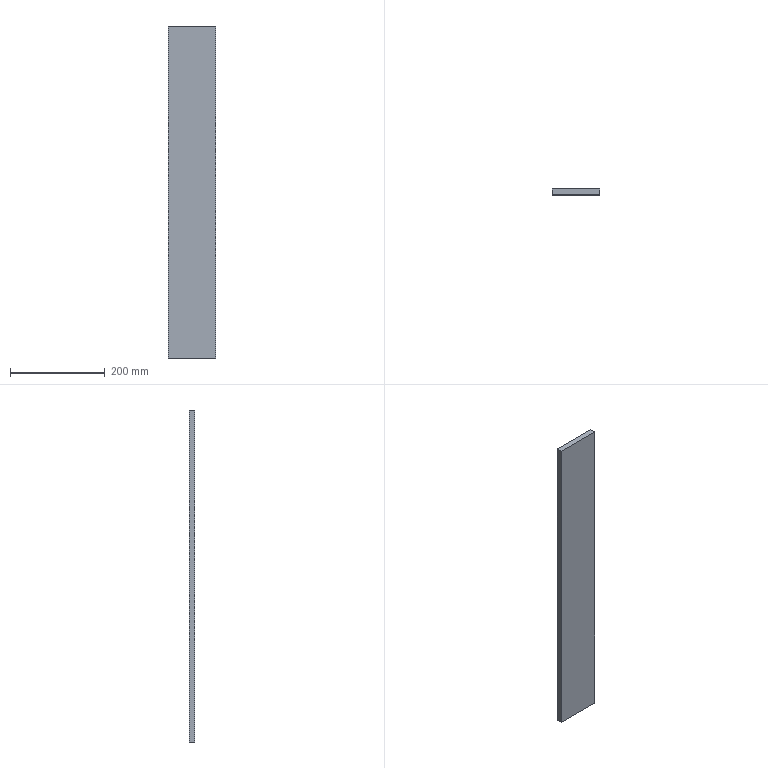Component | NX | CHAPA_INTERNA | 1 solid | 6 faces | box 100 x 12 x 700 mm | volume 840000 mm3 | plane 6
STEP:
#1=CARTESIAN_POINT('',(0.,0.,0.));
#2=DIRECTION('',(0.,0.,1.));
#3=DIRECTION('',(1.,0.,0.));
#4=AXIS2_PLACEMENT_3D('',#1,#2,#3);
#5=CARTESIAN_POINT('',(0.,-22.8,700.));
#6=VERTEX_POINT('',#5);
#7=CARTESIAN_POINT('',(0.,-22.8,0.));
#8=VERTEX_POINT('',#7);
#9=CARTESIAN_POINT('',(0.,-22.8,700.));
#10=DIRECTION('',(0.,0.,-1.));
#11=VECTOR('',#10,1.);
#12=LINE('',#9,#11);
#13=CARTESIAN_POINT('',(0.,-34.8,700.));
#14=DIRECTION('',(1.,0.,0.));
#15=DIRECTION('',(0.,0.,-1.));
#16=AXIS2_PLACEMENT_3D('',#13,#14,#15);
#17=PLANE('',#16);
#18=CARTESIAN_POINT('',(0.,12.));
#19=DIRECTION('',(1.,0.));
#20=VECTOR('',#19,1.);
#21=LINE('',#18,#20);
#22=(GEOMETRIC_REPRESENTATION_CONTEXT(2)PARAMETRIC_REPRESENTATION_CONTEXT()REPRESENTATION_CONTEXT('',''));
#23=DEFINITIONAL_REPRESENTATION('',(#21),#22);
#24=PCURVE('',#17,#23);
#25=CARTESIAN_POINT('',(0.,-22.8,0.));
#26=DIRECTION('',(0.,-1.,0.));
#27=DIRECTION('',(0.,0.,-1.));
#28=AXIS2_PLACEMENT_3D('',#25,#26,#27);
#29=PLANE('',#28);
#30=CARTESIAN_POINT('',(-700.,-0.));
#31=DIRECTION('',(1.,0.));
#32=VECTOR('',#31,1.);
#33=LINE('',#30,#32);
#34=(GEOMETRIC_REPRESENTATION_CONTEXT(2)PARAMETRIC_REPRESENTATION_CONTEXT()REPRESENTATION_CONTEXT('',''));
#35=DEFINITIONAL_REPRESENTATION('',(#33),#34);
#36=PCURVE('',#29,#35);
#37=SURFACE_CURVE('',#12,(#24,#36),.PCURVE_S1.);
#38=EDGE_CURVE('',#6,#8,#37,.T.);
#39=ORIENTED_EDGE('',*,*,#38,.T.);
#40=CARTESIAN_POINT('',(0.,-34.8,0.));
#41=VERTEX_POINT('',#40);
#42=CARTESIAN_POINT('',(0.,-34.8,0.));
#43=DIRECTION('',(0.,1.,0.));
#44=VECTOR('',#43,1.);
#45=LINE('',#42,#44);
#46=CARTESIAN_POINT('',(700.,0.));
#47=DIRECTION('',(0.,1.));
#48=VECTOR('',#47,1.);
#49=LINE('',#46,#48);
#50=(GEOMETRIC_REPRESENTATION_CONTEXT(2)PARAMETRIC_REPRESENTATION_CONTEXT()REPRESENTATION_CONTEXT('',''));
#51=DEFINITIONAL_REPRESENTATION('',(#49),#50);
#52=PCURVE('',#17,#51);
#53=CARTESIAN_POINT('',(0.,-34.8,0.));
#54=DIRECTION('',(-0.,0.,1.));
#55=DIRECTION('',(1.,0.,0.));
#56=AXIS2_PLACEMENT_3D('',#53,#54,#55);
#57=PLANE('',#56);
#58=CARTESIAN_POINT('',(0.,0.));
#59=DIRECTION('',(0.,1.));
#60=VECTOR('',#59,1.);
#61=LINE('',#58,#60);
#62=(GEOMETRIC_REPRESENTATION_CONTEXT(2)PARAMETRIC_REPRESENTATION_CONTEXT()REPRESENTATION_CONTEXT('',''));
#63=DEFINITIONAL_REPRESENTATION('',(#61),#62);
#64=PCURVE('',#57,#63);
#65=SURFACE_CURVE('',#45,(#52,#64),.PCURVE_S1.);
#66=EDGE_CURVE('',#41,#8,#65,.T.);
#67=ORIENTED_EDGE('',*,*,#66,.F.);
#68=CARTESIAN_POINT('',(0.,-34.8,700.));
#69=VERTEX_POINT('',#68);
#70=CARTESIAN_POINT('',(0.,-34.8,700.));
#71=DIRECTION('',(0.,0.,-1.));
#72=VECTOR('',#71,1.);
#73=LINE('',#70,#72);
#74=CARTESIAN_POINT('',(0.,0.));
#75=DIRECTION('',(1.,0.));
#76=VECTOR('',#75,1.);
#77=LINE('',#74,#76);
#78=(GEOMETRIC_REPRESENTATION_CONTEXT(2)PARAMETRIC_REPRESENTATION_CONTEXT()REPRESENTATION_CONTEXT('',''));
#79=DEFINITIONAL_REPRESENTATION('',(#77),#78);
#80=PCURVE('',#17,#79);
#81=CARTESIAN_POINT('',(0.,-34.8,0.));
#82=DIRECTION('',(0.,-1.,0.));
#83=DIRECTION('',(0.,0.,-1.));
#84=AXIS2_PLACEMENT_3D('',#81,#82,#83);
#85=PLANE('',#84);
#86=CARTESIAN_POINT('',(-700.,-0.));
#87=DIRECTION('',(1.,0.));
#88=VECTOR('',#87,1.);
#89=LINE('',#86,#88);
#90=(GEOMETRIC_REPRESENTATION_CONTEXT(2)PARAMETRIC_REPRESENTATION_CONTEXT()REPRESENTATION_CONTEXT('',''));
#91=DEFINITIONAL_REPRESENTATION('',(#89),#90);
#92=PCURVE('',#85,#91);
#93=SURFACE_CURVE('',#73,(#80,#92),.PCURVE_S1.);
#94=EDGE_CURVE('',#69,#41,#93,.T.);
#95=ORIENTED_EDGE('',*,*,#94,.F.);
#96=CARTESIAN_POINT('',(0.,-34.8,700.));
#97=DIRECTION('',(0.,1.,0.));
#98=VECTOR('',#97,1.);
#99=LINE('',#96,#98);
#100=CARTESIAN_POINT('',(0.,0.));
#101=DIRECTION('',(0.,1.));
#102=VECTOR('',#101,1.);
#103=LINE('',#100,#102);
#104=(GEOMETRIC_REPRESENTATION_CONTEXT(2)PARAMETRIC_REPRESENTATION_CONTEXT()REPRESENTATION_CONTEXT('',''));
#105=DEFINITIONAL_REPRESENTATION('',(#103),#104);
#106=PCURVE('',#17,#105);
#107=CARTESIAN_POINT('',(100.,-34.8,700.));
#108=DIRECTION('',(0.,0.,-1.));
#109=DIRECTION('',(-1.,0.,0.));
#110=AXIS2_PLACEMENT_3D('',#107,#108,#109);
#111=PLANE('',#110);
#112=CARTESIAN_POINT('',(100.,0.));
#113=DIRECTION('',(0.,1.));
#114=VECTOR('',#113,1.);
#115=LINE('',#112,#114);
#116=(GEOMETRIC_REPRESENTATION_CONTEXT(2)PARAMETRIC_REPRESENTATION_CONTEXT()REPRESENTATION_CONTEXT('',''));
#117=DEFINITIONAL_REPRESENTATION('',(#115),#116);
#118=PCURVE('',#111,#117);
#119=SURFACE_CURVE('',#99,(#106,#118),.PCURVE_S1.);
#120=EDGE_CURVE('',#69,#6,#119,.T.);
#121=ORIENTED_EDGE('',*,*,#120,.T.);
#122=EDGE_LOOP('',(#39,#67,#95,#121));
#123=FACE_BOUND('',#122,.T.);
#124=ADVANCED_FACE('',(#123),#17,.F.);
#125=CARTESIAN_POINT('',(100.,-22.8,0.));
#126=VERTEX_POINT('',#125);
#127=CARTESIAN_POINT('',(0.,-22.8,0.));
#128=DIRECTION('',(1.,0.,0.));
#129=VECTOR('',#128,1.);
#130=LINE('',#127,#129);
#131=CARTESIAN_POINT('',(0.,12.));
#132=DIRECTION('',(1.,0.));
#133=VECTOR('',#132,1.);
#134=LINE('',#131,#133);
#135=(GEOMETRIC_REPRESENTATION_CONTEXT(2)PARAMETRIC_REPRESENTATION_CONTEXT()REPRESENTATION_CONTEXT('',''));
#136=DEFINITIONAL_REPRESENTATION('',(#134),#135);
#137=PCURVE('',#57,#136);
#138=CARTESIAN_POINT('',(0.,0.));
#139=DIRECTION('',(-0.,1.));
#140=VECTOR('',#139,1.);
#141=LINE('',#138,#140);
#142=(GEOMETRIC_REPRESENTATION_CONTEXT(2)PARAMETRIC_REPRESENTATION_CONTEXT()REPRESENTATION_CONTEXT('',''));
#143=DEFINITIONAL_REPRESENTATION('',(#141),#142);
#144=PCURVE('',#29,#143);
#145=SURFACE_CURVE('',#130,(#137,#144),.PCURVE_S1.);
#146=EDGE_CURVE('',#8,#126,#145,.T.);
#147=ORIENTED_EDGE('',*,*,#146,.T.);
#148=CARTESIAN_POINT('',(100.,-34.8,0.));
#149=VERTEX_POINT('',#148);
#150=CARTESIAN_POINT('',(100.,-34.8,0.));
#151=DIRECTION('',(0.,1.,0.));
#152=VECTOR('',#151,1.);
#153=LINE('',#150,#152);
#154=CARTESIAN_POINT('',(100.,0.));
#155=DIRECTION('',(0.,1.));
#156=VECTOR('',#155,1.);
#157=LINE('',#154,#156);
#158=(GEOMETRIC_REPRESENTATION_CONTEXT(2)PARAMETRIC_REPRESENTATION_CONTEXT()REPRESENTATION_CONTEXT('',''));
#159=DEFINITIONAL_REPRESENTATION('',(#157),#158);
#160=PCURVE('',#57,#159);
#161=CARTESIAN_POINT('',(100.,-34.8,0.));
#162=DIRECTION('',(-1.,0.,-0.));
#163=DIRECTION('',(-0.,0.,1.));
#164=AXIS2_PLACEMENT_3D('',#161,#162,#163);
#165=PLANE('',#164);
#166=CARTESIAN_POINT('',(0.,0.));
#167=DIRECTION('',(0.,1.));
#168=VECTOR('',#167,1.);
#169=LINE('',#166,#168);
#170=(GEOMETRIC_REPRESENTATION_CONTEXT(2)PARAMETRIC_REPRESENTATION_CONTEXT()REPRESENTATION_CONTEXT('',''));
#171=DEFINITIONAL_REPRESENTATION('',(#169),#170);
#172=PCURVE('',#165,#171);
#173=SURFACE_CURVE('',#153,(#160,#172),.PCURVE_S1.);
#174=EDGE_CURVE('',#149,#126,#173,.T.);
#175=ORIENTED_EDGE('',*,*,#174,.F.);
#176=CARTESIAN_POINT('',(0.,-34.8,0.));
#177=DIRECTION('',(1.,0.,0.));
#178=VECTOR('',#177,1.);
#179=LINE('',#176,#178);
#180=CARTESIAN_POINT('',(0.,0.));
#181=DIRECTION('',(1.,0.));
#182=VECTOR('',#181,1.);
#183=LINE('',#180,#182);
#184=(GEOMETRIC_REPRESENTATION_CONTEXT(2)PARAMETRIC_REPRESENTATION_CONTEXT()REPRESENTATION_CONTEXT('',''));
#185=DEFINITIONAL_REPRESENTATION('',(#183),#184);
#186=PCURVE('',#57,#185);
#187=CARTESIAN_POINT('',(0.,0.));
#188=DIRECTION('',(-0.,1.));
#189=VECTOR('',#188,1.);
#190=LINE('',#187,#189);
#191=(GEOMETRIC_REPRESENTATION_CONTEXT(2)PARAMETRIC_REPRESENTATION_CONTEXT()REPRESENTATION_CONTEXT('',''));
#192=DEFINITIONAL_REPRESENTATION('',(#190),#191);
#193=PCURVE('',#85,#192);
#194=SURFACE_CURVE('',#179,(#186,#193),.PCURVE_S1.);
#195=EDGE_CURVE('',#41,#149,#194,.T.);
#196=ORIENTED_EDGE('',*,*,#195,.F.);
#197=ORIENTED_EDGE('',*,*,#66,.T.);
#198=EDGE_LOOP('',(#147,#175,#196,#197));
#199=FACE_BOUND('',#198,.T.);
#200=ADVANCED_FACE('',(#199),#57,.F.);
#201=CARTESIAN_POINT('',(100.,-22.8,700.));
#202=VERTEX_POINT('',#201);
#203=CARTESIAN_POINT('',(100.,-22.8,0.));
#204=DIRECTION('',(-0.,0.,1.));
#205=VECTOR('',#204,1.);
#206=LINE('',#203,#205);
#207=CARTESIAN_POINT('',(0.,12.));
#208=DIRECTION('',(1.,0.));
#209=VECTOR('',#208,1.);
#210=LINE('',#207,#209);
#211=(GEOMETRIC_REPRESENTATION_CONTEXT(2)PARAMETRIC_REPRESENTATION_CONTEXT()REPRESENTATION_CONTEXT('',''));
#212=DEFINITIONAL_REPRESENTATION('',(#210),#211);
#213=PCURVE('',#165,#212);
#214=CARTESIAN_POINT('',(0.,100.));
#215=DIRECTION('',(-1.,-0.));
#216=VECTOR('',#215,1.);
#217=LINE('',#214,#216);
#218=(GEOMETRIC_REPRESENTATION_CONTEXT(2)PARAMETRIC_REPRESENTATION_CONTEXT()REPRESENTATION_CONTEXT('',''));
#219=DEFINITIONAL_REPRESENTATION('',(#217),#218);
#220=PCURVE('',#29,#219);
#221=SURFACE_CURVE('',#206,(#213,#220),.PCURVE_S1.);
#222=EDGE_CURVE('',#126,#202,#221,.T.);
#223=ORIENTED_EDGE('',*,*,#222,.T.);
#224=CARTESIAN_POINT('',(100.,-34.8,700.));
#225=VERTEX_POINT('',#224);
#226=CARTESIAN_POINT('',(100.,-34.8,700.));
#227=DIRECTION('',(0.,1.,0.));
#228=VECTOR('',#227,1.);
#229=LINE('',#226,#228);
#230=CARTESIAN_POINT('',(700.,0.));
#231=DIRECTION('',(0.,1.));
#232=VECTOR('',#231,1.);
#233=LINE('',#230,#232);
#234=(GEOMETRIC_REPRESENTATION_CONTEXT(2)PARAMETRIC_REPRESENTATION_CONTEXT()REPRESENTATION_CONTEXT('',''));
#235=DEFINITIONAL_REPRESENTATION('',(#233),#234);
#236=PCURVE('',#165,#235);
#237=CARTESIAN_POINT('',(0.,0.));
#238=DIRECTION('',(0.,1.));
#239=VECTOR('',#238,1.);
#240=LINE('',#237,#239);
#241=(GEOMETRIC_REPRESENTATION_CONTEXT(2)PARAMETRIC_REPRESENTATION_CONTEXT()REPRESENTATION_CONTEXT('',''));
#242=DEFINITIONAL_REPRESENTATION('',(#240),#241);
#243=PCURVE('',#111,#242);
#244=SURFACE_CURVE('',#229,(#236,#243),.PCURVE_S1.);
#245=EDGE_CURVE('',#225,#202,#244,.T.);
#246=ORIENTED_EDGE('',*,*,#245,.F.);
#247=CARTESIAN_POINT('',(100.,-34.8,0.));
#248=DIRECTION('',(-0.,0.,1.));
#249=VECTOR('',#248,1.);
#250=LINE('',#247,#249);
#251=CARTESIAN_POINT('',(0.,0.));
#252=DIRECTION('',(1.,0.));
#253=VECTOR('',#252,1.);
#254=LINE('',#251,#253);
#255=(GEOMETRIC_REPRESENTATION_CONTEXT(2)PARAMETRIC_REPRESENTATION_CONTEXT()REPRESENTATION_CONTEXT('',''));
#256=DEFINITIONAL_REPRESENTATION('',(#254),#255);
#257=PCURVE('',#165,#256);
#258=CARTESIAN_POINT('',(0.,100.));
#259=DIRECTION('',(-1.,-0.));
#260=VECTOR('',#259,1.);
#261=LINE('',#258,#260);
#262=(GEOMETRIC_REPRESENTATION_CONTEXT(2)PARAMETRIC_REPRESENTATION_CONTEXT()REPRESENTATION_CONTEXT('',''));
#263=DEFINITIONAL_REPRESENTATION('',(#261),#262);
#264=PCURVE('',#85,#263);
#265=SURFACE_CURVE('',#250,(#257,#264),.PCURVE_S1.);
#266=EDGE_CURVE('',#149,#225,#265,.T.);
#267=ORIENTED_EDGE('',*,*,#266,.F.);
#268=ORIENTED_EDGE('',*,*,#174,.T.);
#269=EDGE_LOOP('',(#223,#246,#267,#268));
#270=FACE_BOUND('',#269,.T.);
#271=ADVANCED_FACE('',(#270),#165,.F.);
#272=CARTESIAN_POINT('',(100.,-22.8,700.));
#273=DIRECTION('',(-1.,0.,0.));
#274=VECTOR('',#273,1.);
#275=LINE('',#272,#274);
#276=CARTESIAN_POINT('',(0.,12.));
#277=DIRECTION('',(1.,0.));
#278=VECTOR('',#277,1.);
#279=LINE('',#276,#278);
#280=(GEOMETRIC_REPRESENTATION_CONTEXT(2)PARAMETRIC_REPRESENTATION_CONTEXT()REPRESENTATION_CONTEXT('',''));
#281=DEFINITIONAL_REPRESENTATION('',(#279),#280);
#282=PCURVE('',#111,#281);
#283=CARTESIAN_POINT('',(-700.,100.));
#284=DIRECTION('',(0.,-1.));
#285=VECTOR('',#284,1.);
#286=LINE('',#283,#285);
#287=(GEOMETRIC_REPRESENTATION_CONTEXT(2)PARAMETRIC_REPRESENTATION_CONTEXT()REPRESENTATION_CONTEXT('',''));
#288=DEFINITIONAL_REPRESENTATION('',(#286),#287);
#289=PCURVE('',#29,#288);
#290=SURFACE_CURVE('',#275,(#282,#289),.PCURVE_S1.);
#291=EDGE_CURVE('',#202,#6,#290,.T.);
#292=ORIENTED_EDGE('',*,*,#291,.T.);
#293=ORIENTED_EDGE('',*,*,#120,.F.);
#294=CARTESIAN_POINT('',(100.,-34.8,700.));
#295=DIRECTION('',(-1.,0.,0.));
#296=VECTOR('',#295,1.);
#297=LINE('',#294,#296);
#298=CARTESIAN_POINT('',(0.,0.));
#299=DIRECTION('',(1.,0.));
#300=VECTOR('',#299,1.);
#301=LINE('',#298,#300);
#302=(GEOMETRIC_REPRESENTATION_CONTEXT(2)PARAMETRIC_REPRESENTATION_CONTEXT()REPRESENTATION_CONTEXT('',''));
#303=DEFINITIONAL_REPRESENTATION('',(#301),#302);
#304=PCURVE('',#111,#303);
#305=CARTESIAN_POINT('',(-700.,100.));
#306=DIRECTION('',(0.,-1.));
#307=VECTOR('',#306,1.);
#308=LINE('',#305,#307);
#309=(GEOMETRIC_REPRESENTATION_CONTEXT(2)PARAMETRIC_REPRESENTATION_CONTEXT()REPRESENTATION_CONTEXT('',''));
#310=DEFINITIONAL_REPRESENTATION('',(#308),#309);
#311=PCURVE('',#85,#310);
#312=SURFACE_CURVE('',#297,(#304,#311),.PCURVE_S1.);
#313=EDGE_CURVE('',#225,#69,#312,.T.);
#314=ORIENTED_EDGE('',*,*,#313,.F.);
#315=ORIENTED_EDGE('',*,*,#245,.T.);
#316=EDGE_LOOP('',(#292,#293,#314,#315));
#317=FACE_BOUND('',#316,.T.);
#318=ADVANCED_FACE('',(#317),#111,.F.);
#319=ORIENTED_EDGE('',*,*,#94,.T.);
#320=ORIENTED_EDGE('',*,*,#195,.T.);
#321=ORIENTED_EDGE('',*,*,#266,.T.);
#322=ORIENTED_EDGE('',*,*,#313,.T.);
#323=EDGE_LOOP('',(#319,#320,#321,#322));
#324=FACE_BOUND('',#323,.T.);
#325=ADVANCED_FACE('',(#324),#85,.T.);
#326=ORIENTED_EDGE('',*,*,#38,.F.);
#327=ORIENTED_EDGE('',*,*,#291,.F.);
#328=ORIENTED_EDGE('',*,*,#222,.F.);
#329=ORIENTED_EDGE('',*,*,#146,.F.);
#330=EDGE_LOOP('',(#326,#327,#328,#329));
#331=FACE_BOUND('',#330,.T.);
#332=ADVANCED_FACE('',(#331),#29,.F.);
#333=CLOSED_SHELL('',(#124,#200,#271,#318,#325,#332));
#334=MANIFOLD_SOLID_BREP('',#333);
#335=(LENGTH_UNIT()NAMED_UNIT(*)SI_UNIT(.MILLI.,.METRE.));
#336=UNCERTAINTY_MEASURE_WITH_UNIT(LENGTH_MEASURE(0.0000001),#335,'','');
#337=(NAMED_UNIT(*)PLANE_ANGLE_UNIT()SI_UNIT($,.RADIAN.));
#338=(NAMED_UNIT(*)SI_UNIT($,.STERADIAN.)SOLID_ANGLE_UNIT());
#339=(GEOMETRIC_REPRESENTATION_CONTEXT(3)GLOBAL_UNCERTAINTY_ASSIGNED_CONTEXT((#336))GLOBAL_UNIT_ASSIGNED_CONTEXT((#335,#337,#338))REPRESENTATION_CONTEXT('',''));
#340=ADVANCED_BREP_SHAPE_REPRESENTATION('',(#4,#334),#339);